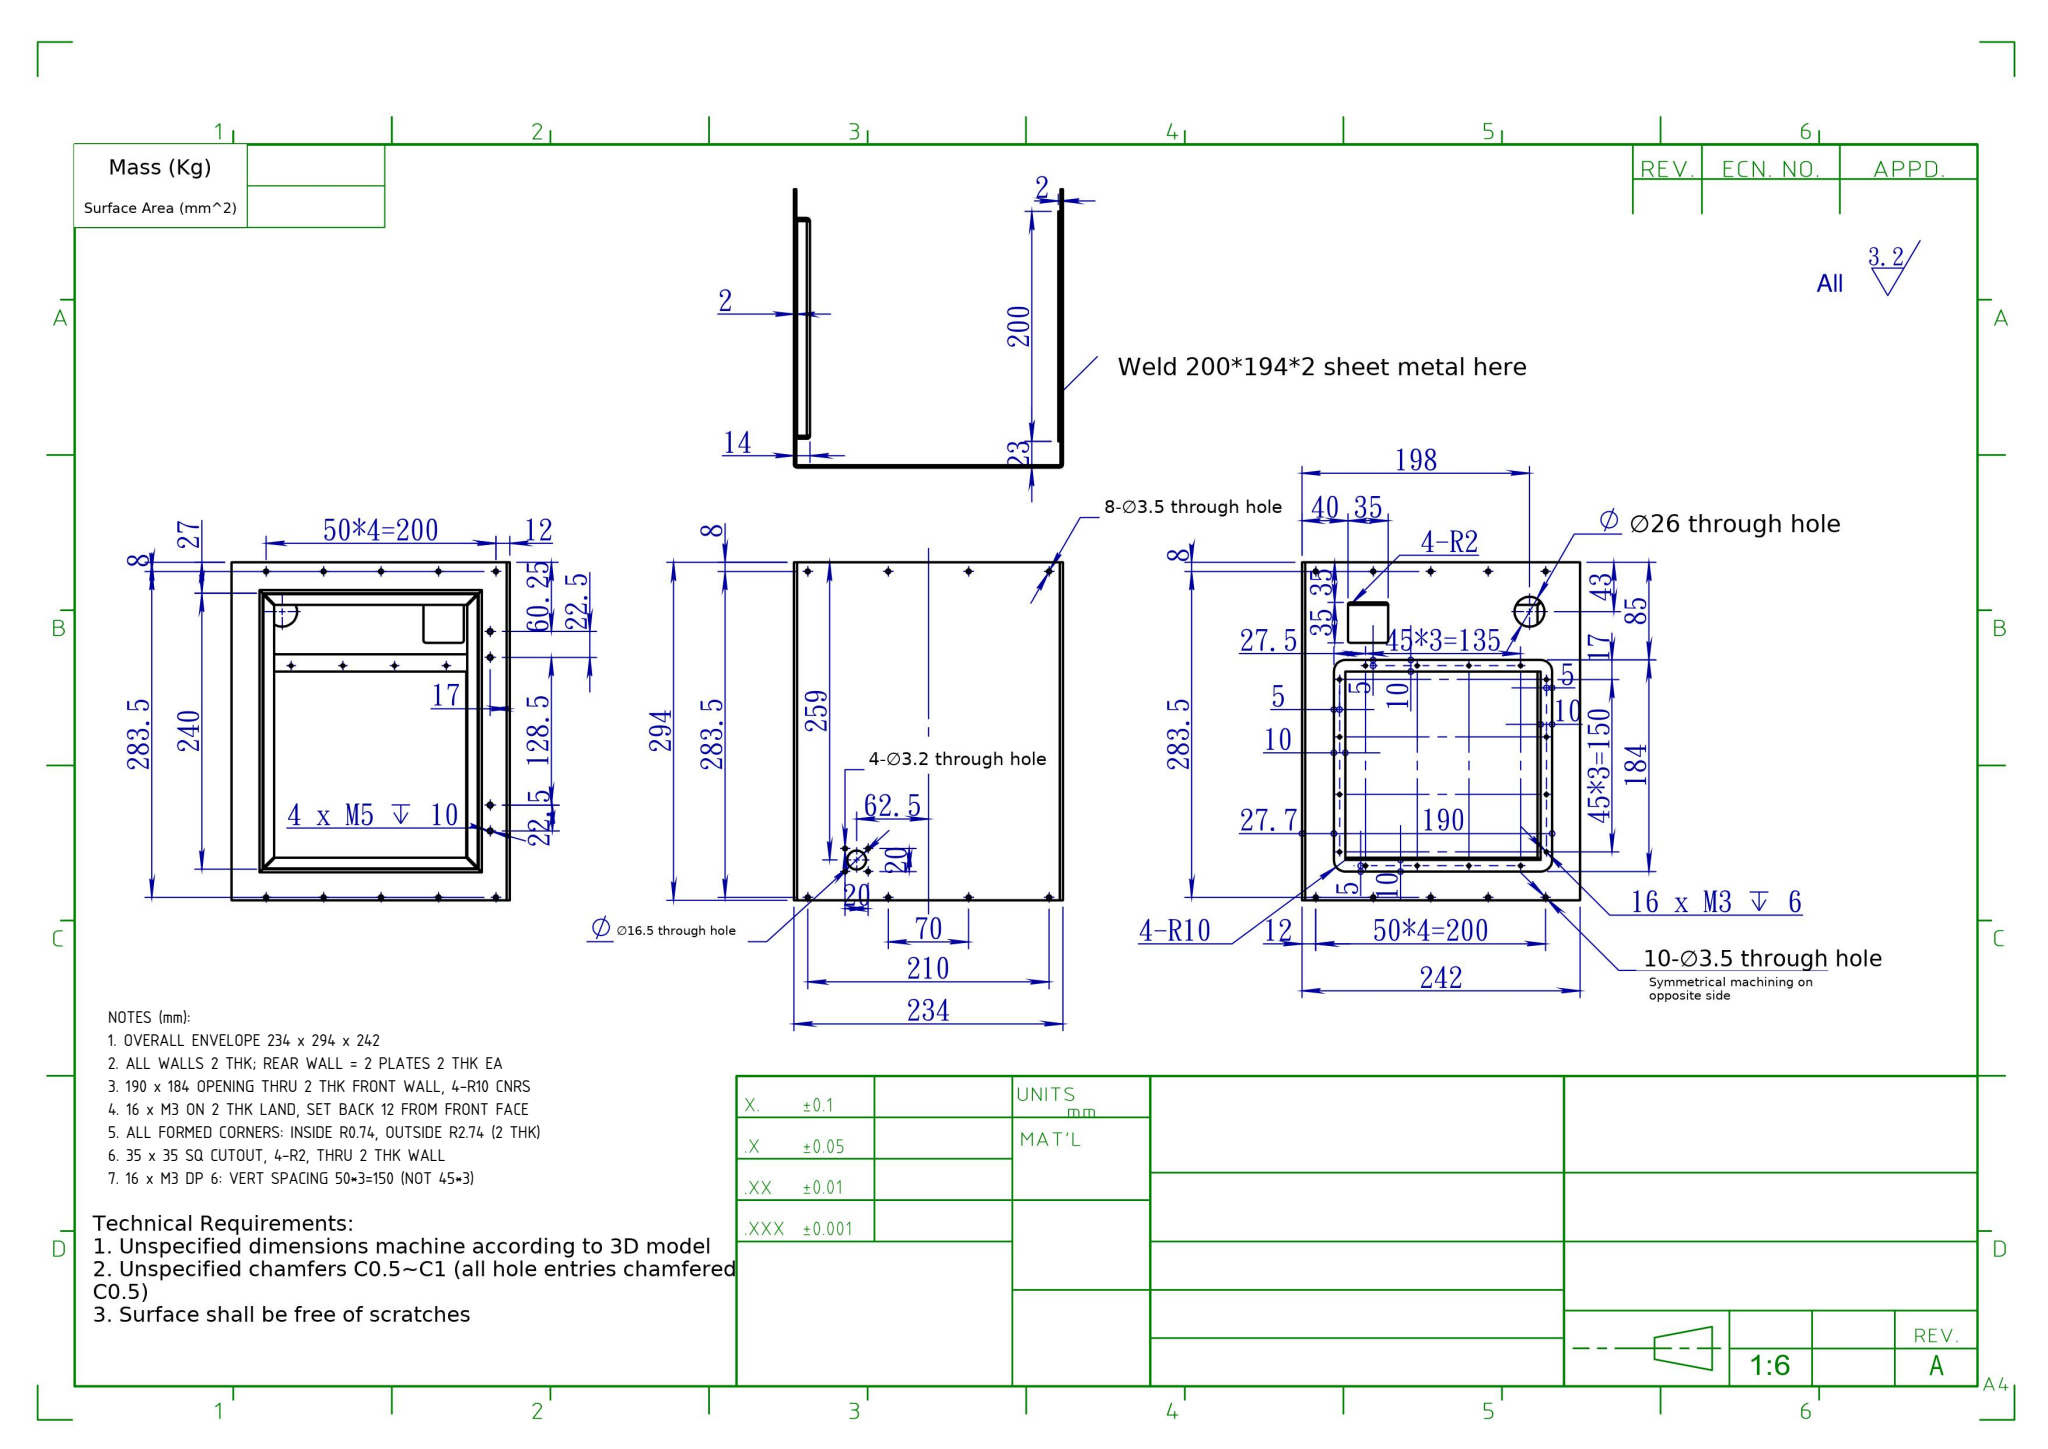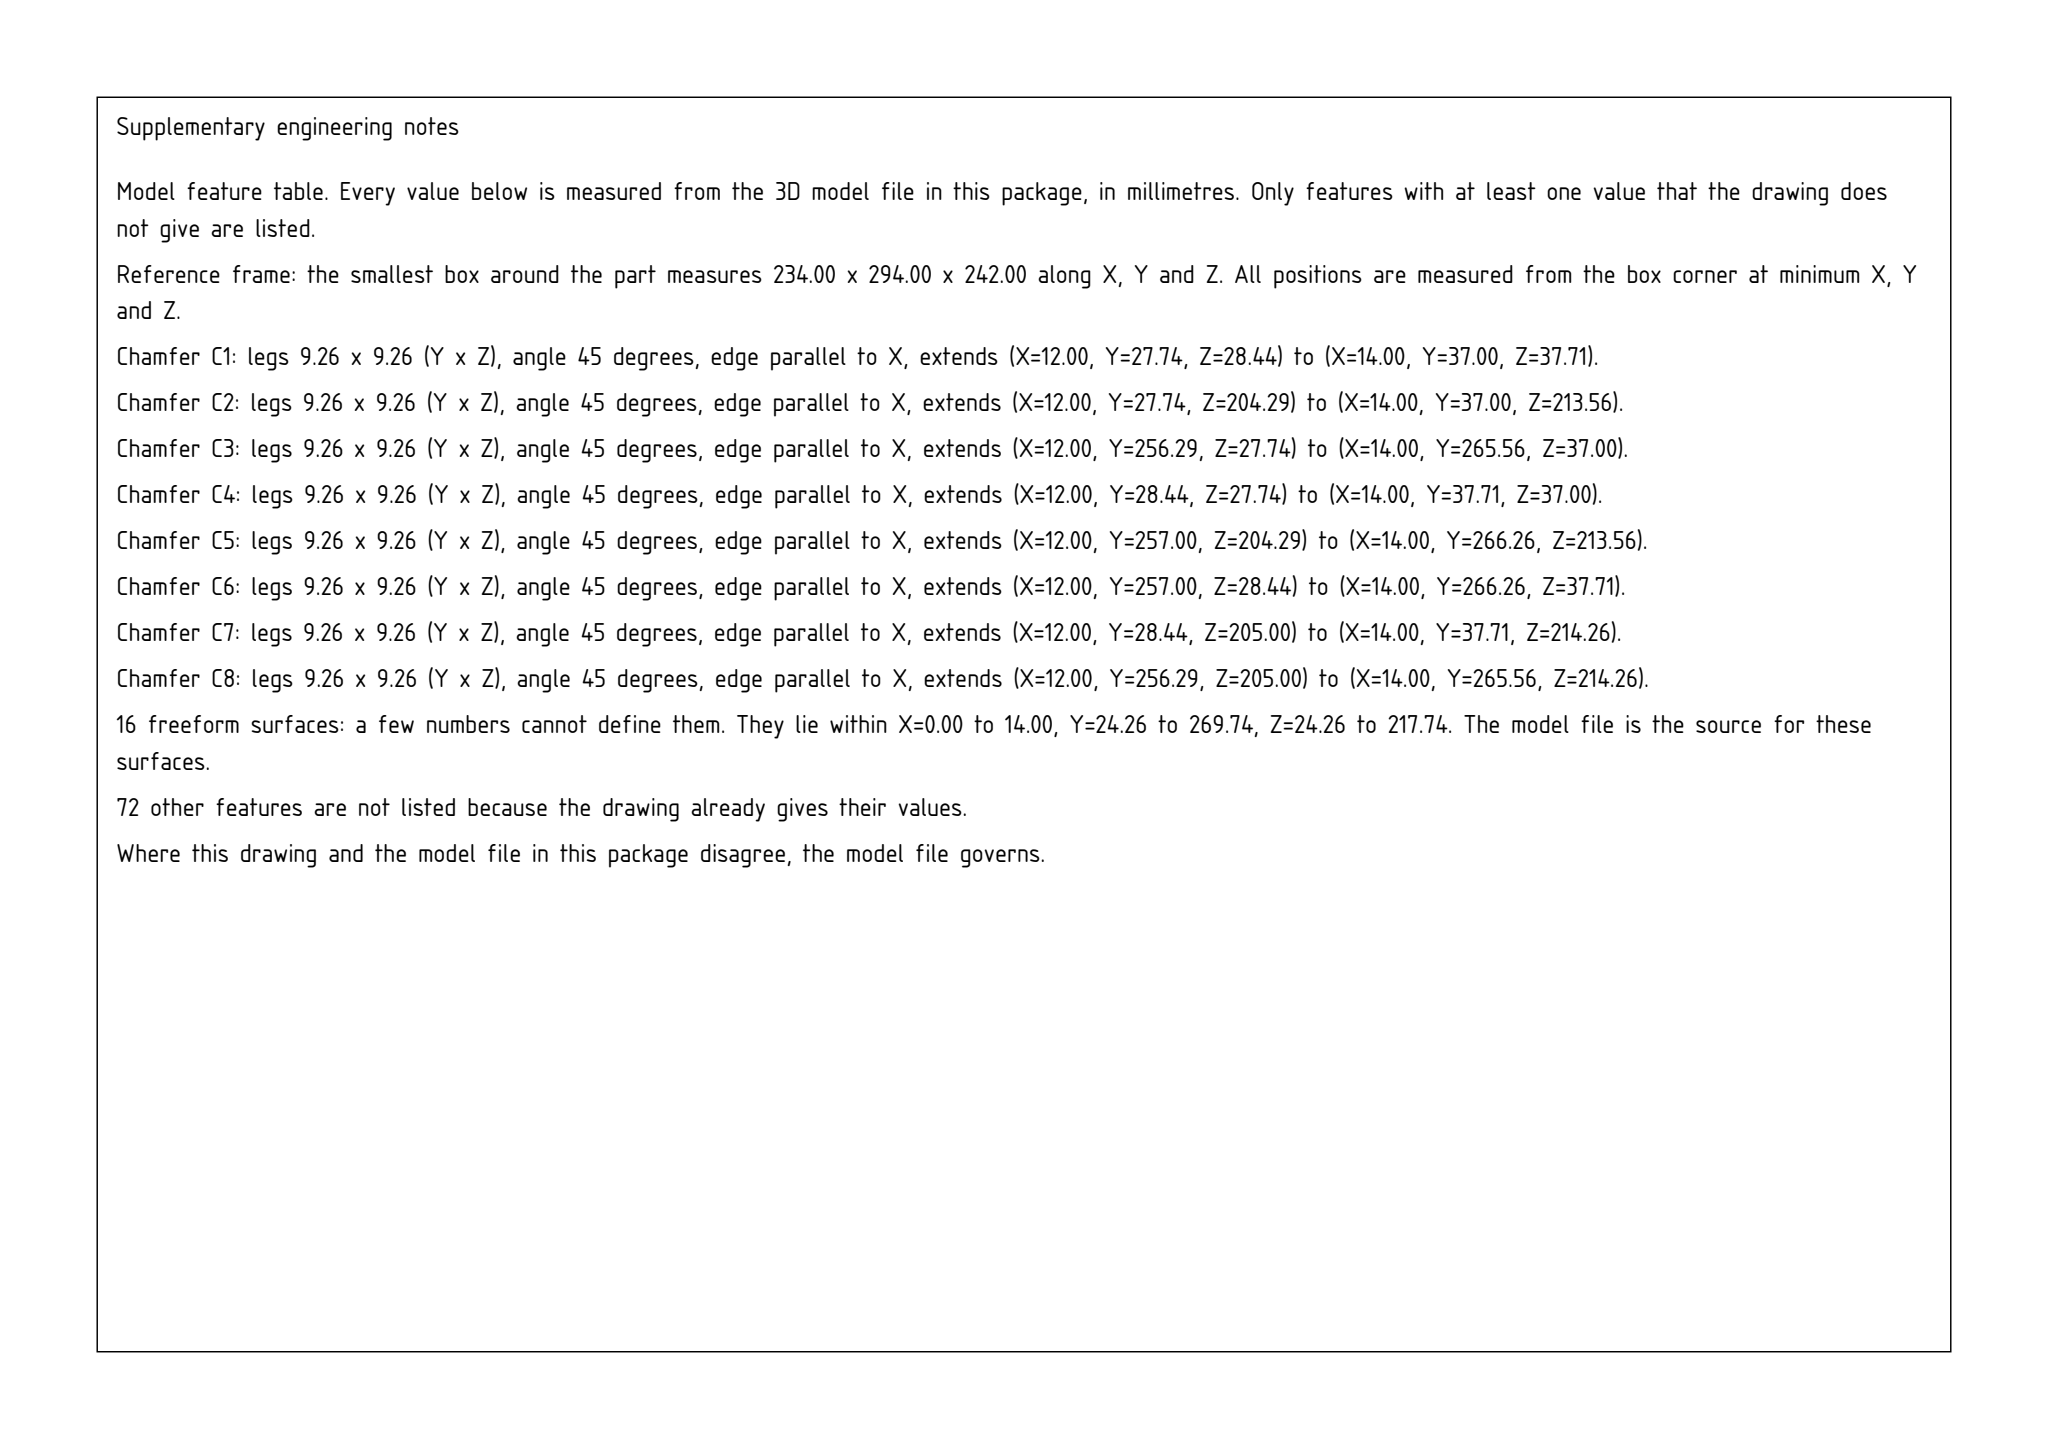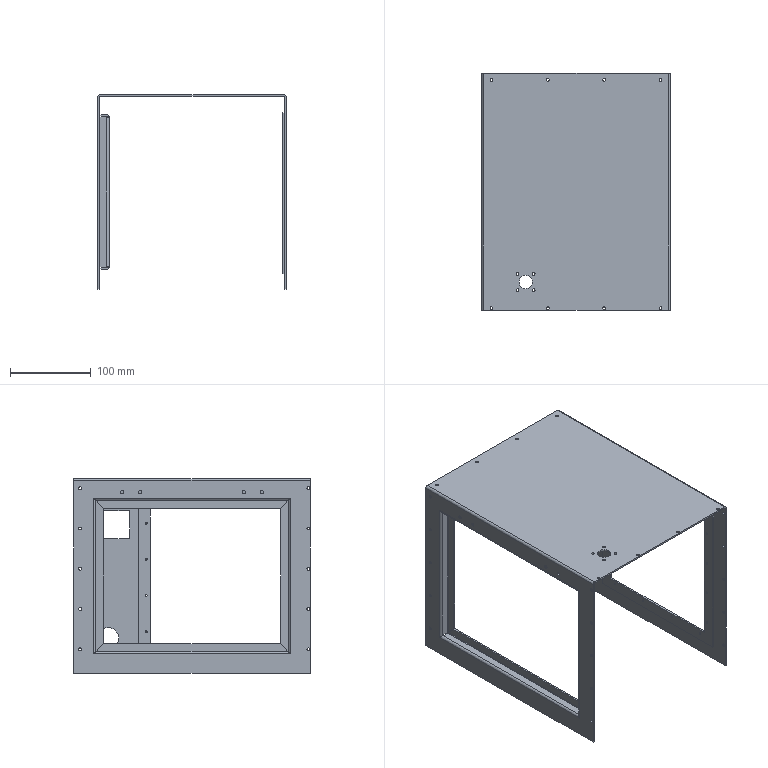Part | SolidWorks | mm | 1 solid | 224 faces | box 234 x 294 x 242 mm | volume 310056 mm3 | cylinder 136 | plane 72 | spline 16 | commonest cylinder face diameters 3.5 x56 2.5 x32 5.473 x10 1.473 x10 4.2 x8 3.2 x8 4 x4 20 x4
Drawing notes:
OVERALL ENVELOPE 234 x 294 x 242 | from the solid: bbox_xyz 234.02 x 294.0 x 242.0
ALL WALLS 2 THK; REAR WALL = 2 PLATES 2 THK EA | from the solid: x planes 0.02/2.02, 12.02/14.02, 230.02/232.02, 232.02/234.02 (232.02 count 2 = two coincident plate faces)
190 x 184 OPENING THRU 2 THK FRONT WALL, 4-R10 CNRS | from the solid: Ø20 corner cyls (R10) at y35/199, z34.26/204.26 len 2.0; faces x=0.02/2.02; opening z24.26-214.26 x y25-209
16 x M3 ON 2 THK LAND, SET BACK 12 FROM FRONT FACE | from the solid: Ø2.5 x-axis holes len 2.0 in plate bounded by x=12.02 and x=14.02; front outer face x=0.02 -> 12.00 setback
ALL FORMED CORNERS: INSIDE R0.74, OUTSIDE R2.74 (2 THK) | from the solid: Corner cylinders dia 1.473 (R0.736) inside & dia 5.473 (R2.736) outside, axes Y and Z along all four 2 mm wall junctions
35 x 35 SQ CUTOUT, 4-R2, THRU 2 THK WALL | from the solid: Cutout bounded by planes y=224/259 and z=167/202 (35x35) in wall between x=12.02 and x=14.02 (2 thk), same wall as Ø26 x 2.0 thru hole
16 x M3 DP 6: VERT SPACING 50*3=150 (NOT 45*3) | from the solid: M3 tap-drill Ø2.5 x 2.0 holes at y=42, 92, 142, 192 => 50 pitch, 3 spaces = 150; horiz z=51.76/96.76/141.76/186.76 => 45 pitch